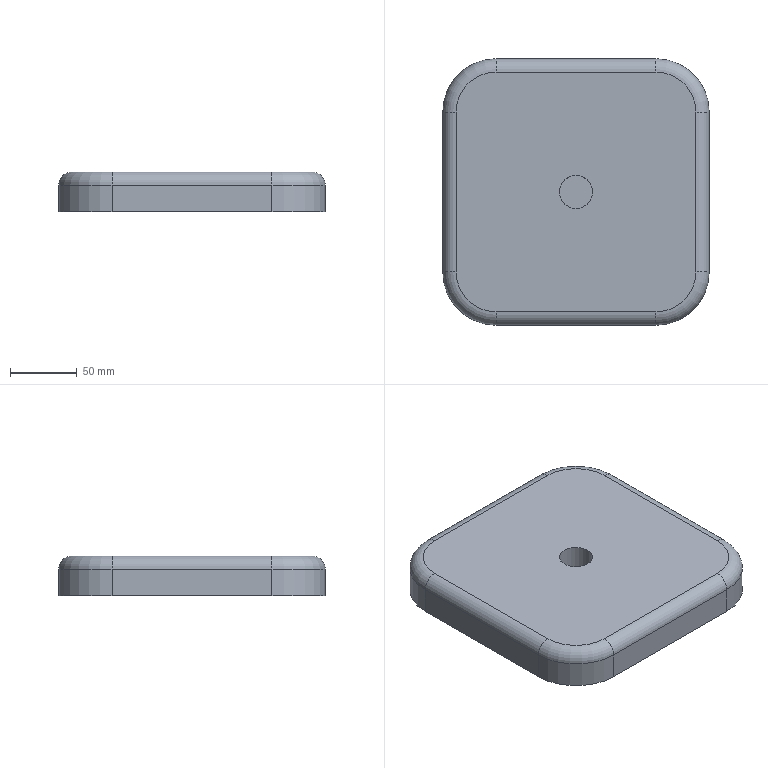Component | NX | BASE | 1 solid | 20 faces | volume 1133586 mm3 | cylinder 9 | plane 7 | torus 4 | commonest cylinder face diameters 80 x4 20 x4 25 x1